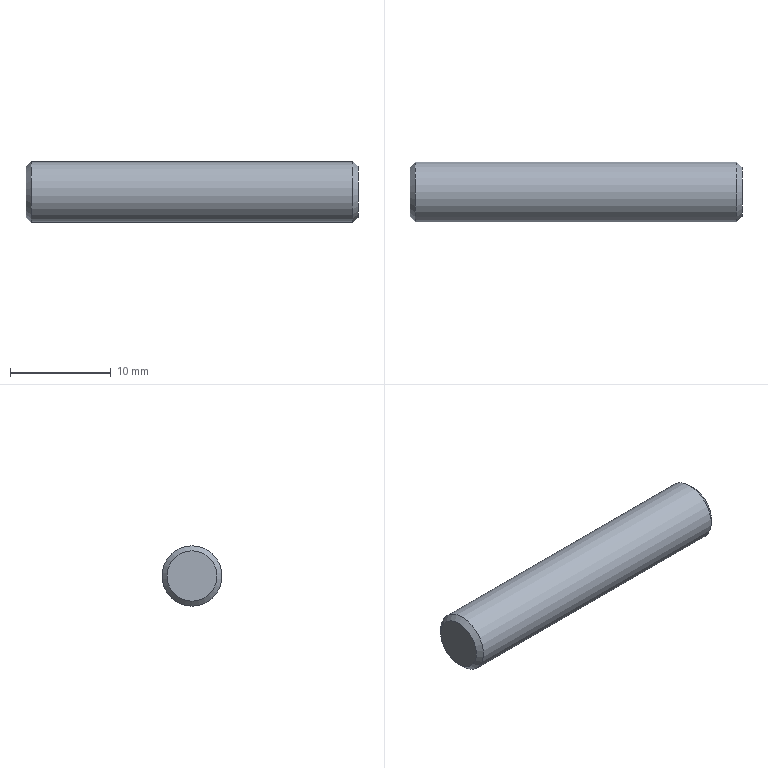Component | NX | STUD | 1 solid | 5 faces | box 33 x 6 x 6 mm | volume 929 mm3 | plane 2 | cone 2 | cylinder 1 | commonest cylinder face diameters 6 x1
STEP:
#1=CARTESIAN_POINT('',(0.,0.,0.));
#2=DIRECTION('',(0.,0.,1.));
#3=DIRECTION('',(1.,0.,0.));
#4=AXIS2_PLACEMENT_3D('',#1,#2,#3);
#5=CARTESIAN_POINT('',(-36.268,-25.,7.));
#6=VERTEX_POINT('',#5);
#7=CARTESIAN_POINT('',(-36.268,-25.,9.5));
#8=DIRECTION('',(1.,0.,0.));
#9=DIRECTION('',(0.,0.,-1.));
#10=AXIS2_PLACEMENT_3D('',#7,#8,#9);
#11=CIRCLE('',#10,2.5);
#12=CARTESIAN_POINT('',(-36.268,-25.,9.5));
#13=DIRECTION('',(1.,0.,0.));
#14=DIRECTION('',(0.,0.,-1.));
#15=AXIS2_PLACEMENT_3D('',#12,#13,#14);
#16=PLANE('',#15);
#17=CARTESIAN_POINT('',(0.,0.));
#18=DIRECTION('',(1.,0.));
#19=AXIS2_PLACEMENT_2D('',#17,#18);
#20=CIRCLE('',#19,2.5);
#21=(GEOMETRIC_REPRESENTATION_CONTEXT(2)PARAMETRIC_REPRESENTATION_CONTEXT()REPRESENTATION_CONTEXT('',''));
#22=DEFINITIONAL_REPRESENTATION('',(#20),#21);
#23=PCURVE('',#16,#22);
#24=CARTESIAN_POINT('',(-36.768,-25.,9.5));
#25=DIRECTION('',(-1.,0.,0.));
#26=DIRECTION('',(0.,0.,1.));
#27=AXIS2_PLACEMENT_3D('',#24,#25,#26);
#28=CONICAL_SURFACE('',#27,3.,0.7854);
#29=CARTESIAN_POINT('',(9.425,-0.5));
#30=DIRECTION('',(-1.,0.));
#31=VECTOR('',#30,1.);
#32=LINE('',#29,#31);
#33=(GEOMETRIC_REPRESENTATION_CONTEXT(2)PARAMETRIC_REPRESENTATION_CONTEXT()REPRESENTATION_CONTEXT('',''));
#34=DEFINITIONAL_REPRESENTATION('',(#32),#33);
#35=PCURVE('',#28,#34);
#36=SURFACE_CURVE('',#11,(#23,#35),.PCURVE_S1.);
#37=EDGE_CURVE('',#6,#6,#36,.T.);
#38=ORIENTED_EDGE('',*,*,#37,.T.);
#39=EDGE_LOOP('',(#38));
#40=FACE_BOUND('',#39,.T.);
#41=ADVANCED_FACE('',(#40),#16,.T.);
#42=CARTESIAN_POINT('',(-69.268,-25.,12.));
#43=VERTEX_POINT('',#42);
#44=CARTESIAN_POINT('',(-69.268,-25.,9.5));
#45=DIRECTION('',(-1.,0.,0.));
#46=DIRECTION('',(0.,0.,1.));
#47=AXIS2_PLACEMENT_3D('',#44,#45,#46);
#48=CIRCLE('',#47,2.5);
#49=CARTESIAN_POINT('',(-69.268,-25.,9.5));
#50=DIRECTION('',(-1.,0.,0.));
#51=DIRECTION('',(0.,0.,1.));
#52=AXIS2_PLACEMENT_3D('',#49,#50,#51);
#53=PLANE('',#52);
#54=CARTESIAN_POINT('',(0.,0.));
#55=DIRECTION('',(1.,0.));
#56=AXIS2_PLACEMENT_2D('',#54,#55);
#57=CIRCLE('',#56,2.5);
#58=(GEOMETRIC_REPRESENTATION_CONTEXT(2)PARAMETRIC_REPRESENTATION_CONTEXT()REPRESENTATION_CONTEXT('',''));
#59=DEFINITIONAL_REPRESENTATION('',(#57),#58);
#60=PCURVE('',#53,#59);
#61=CARTESIAN_POINT('',(-68.768,-25.,9.5));
#62=DIRECTION('',(1.,0.,0.));
#63=DIRECTION('',(0.,0.,-1.));
#64=AXIS2_PLACEMENT_3D('',#61,#62,#63);
#65=CONICAL_SURFACE('',#64,3.,0.7854);
#66=CARTESIAN_POINT('',(9.425,-0.5));
#67=DIRECTION('',(-1.,0.));
#68=VECTOR('',#67,1.);
#69=LINE('',#66,#68);
#70=(GEOMETRIC_REPRESENTATION_CONTEXT(2)PARAMETRIC_REPRESENTATION_CONTEXT()REPRESENTATION_CONTEXT('',''));
#71=DEFINITIONAL_REPRESENTATION('',(#69),#70);
#72=PCURVE('',#65,#71);
#73=SURFACE_CURVE('',#48,(#60,#72),.PCURVE_S1.);
#74=EDGE_CURVE('',#43,#43,#73,.T.);
#75=ORIENTED_EDGE('',*,*,#74,.T.);
#76=EDGE_LOOP('',(#75));
#77=FACE_BOUND('',#76,.T.);
#78=ADVANCED_FACE('',(#77),#53,.T.);
#79=CARTESIAN_POINT('',(-68.768,-25.,12.5));
#80=VERTEX_POINT('',#79);
#81=CARTESIAN_POINT('',(-68.768,-25.,6.5));
#82=VERTEX_POINT('',#81);
#83=CARTESIAN_POINT('',(-68.768,-25.,9.5));
#84=DIRECTION('',(1.,0.,0.));
#85=DIRECTION('',(0.,0.,1.));
#86=AXIS2_PLACEMENT_3D('',#83,#84,#85);
#87=CIRCLE('',#86,3.);
#88=CARTESIAN_POINT('',(-69.268,-25.,9.5));
#89=DIRECTION('',(1.,0.,0.));
#90=DIRECTION('',(0.,0.,-1.));
#91=AXIS2_PLACEMENT_3D('',#88,#89,#90);
#92=CYLINDRICAL_SURFACE('',#91,3.);
#93=CARTESIAN_POINT('',(3.142,0.5));
#94=DIRECTION('',(1.,0.));
#95=VECTOR('',#94,1.);
#96=LINE('',#93,#95);
#97=(GEOMETRIC_REPRESENTATION_CONTEXT(2)PARAMETRIC_REPRESENTATION_CONTEXT()REPRESENTATION_CONTEXT('',''));
#98=DEFINITIONAL_REPRESENTATION('',(#96),#97);
#99=PCURVE('',#92,#98);
#100=CARTESIAN_POINT('',(3.142,0.));
#101=DIRECTION('',(1.,0.));
#102=VECTOR('',#101,1.);
#103=LINE('',#100,#102);
#104=(GEOMETRIC_REPRESENTATION_CONTEXT(2)PARAMETRIC_REPRESENTATION_CONTEXT()REPRESENTATION_CONTEXT('',''));
#105=DEFINITIONAL_REPRESENTATION('',(#103),#104);
#106=PCURVE('',#65,#105);
#107=SURFACE_CURVE('',#87,(#99,#106),.PCURVE_S1.);
#108=EDGE_CURVE('',#80,#82,#107,.T.);
#109=ORIENTED_EDGE('',*,*,#108,.T.);
#110=CARTESIAN_POINT('',(-36.768,-25.,6.5));
#111=VERTEX_POINT('',#110);
#112=CARTESIAN_POINT('',(-68.768,-25.,6.5));
#113=CARTESIAN_POINT('',(-36.768,-25.,6.5));
#114=B_SPLINE_CURVE_WITH_KNOTS('',1,(#112,#113),.UNSPECIFIED.,.F.,.F.,(2,2),(0.5,32.5),.PIECEWISE_BEZIER_KNOTS.);
#115=CARTESIAN_POINT('',(6.283,0.));
#116=DIRECTION('',(0.,1.));
#117=VECTOR('',#116,1.);
#118=LINE('',#115,#117);
#119=(GEOMETRIC_REPRESENTATION_CONTEXT(2)PARAMETRIC_REPRESENTATION_CONTEXT()REPRESENTATION_CONTEXT('',''));
#120=DEFINITIONAL_REPRESENTATION('',(#118),#119);
#121=PCURVE('',#92,#120);
#122=CARTESIAN_POINT('',(0.,0.));
#123=DIRECTION('',(0.,1.));
#124=VECTOR('',#123,1.);
#125=LINE('',#122,#124);
#126=(GEOMETRIC_REPRESENTATION_CONTEXT(2)PARAMETRIC_REPRESENTATION_CONTEXT()REPRESENTATION_CONTEXT('',''));
#127=DEFINITIONAL_REPRESENTATION('',(#125),#126);
#128=PCURVE('',#92,#127);
#129=SEAM_CURVE('',#114,(#121,#128),.PCURVE_S1.);
#130=EDGE_CURVE('',#82,#111,#129,.T.);
#131=ORIENTED_EDGE('',*,*,#130,.T.);
#132=CARTESIAN_POINT('',(-36.768,-25.,9.5));
#133=DIRECTION('',(-1.,0.,0.));
#134=DIRECTION('',(0.,0.,-1.));
#135=AXIS2_PLACEMENT_3D('',#132,#133,#134);
#136=CIRCLE('',#135,3.);
#137=CARTESIAN_POINT('',(6.283,32.5));
#138=DIRECTION('',(-1.,0.));
#139=VECTOR('',#138,1.);
#140=LINE('',#137,#139);
#141=(GEOMETRIC_REPRESENTATION_CONTEXT(2)PARAMETRIC_REPRESENTATION_CONTEXT()REPRESENTATION_CONTEXT('',''));
#142=DEFINITIONAL_REPRESENTATION('',(#140),#141);
#143=PCURVE('',#92,#142);
#144=CARTESIAN_POINT('',(3.142,0.));
#145=DIRECTION('',(1.,0.));
#146=VECTOR('',#145,1.);
#147=LINE('',#144,#146);
#148=(GEOMETRIC_REPRESENTATION_CONTEXT(2)PARAMETRIC_REPRESENTATION_CONTEXT()REPRESENTATION_CONTEXT('',''));
#149=DEFINITIONAL_REPRESENTATION('',(#147),#148);
#150=PCURVE('',#28,#149);
#151=SURFACE_CURVE('',#136,(#143,#150),.PCURVE_S1.);
#152=EDGE_CURVE('',#111,#111,#151,.T.);
#153=ORIENTED_EDGE('',*,*,#152,.T.);
#154=ORIENTED_EDGE('',*,*,#130,.F.);
#155=CARTESIAN_POINT('',(-68.768,-25.,9.5));
#156=DIRECTION('',(1.,0.,0.));
#157=DIRECTION('',(0.,0.,1.));
#158=AXIS2_PLACEMENT_3D('',#155,#156,#157);
#159=CIRCLE('',#158,3.);
#160=CARTESIAN_POINT('',(-3.142,0.5));
#161=DIRECTION('',(1.,0.));
#162=VECTOR('',#161,1.);
#163=LINE('',#160,#162);
#164=(GEOMETRIC_REPRESENTATION_CONTEXT(2)PARAMETRIC_REPRESENTATION_CONTEXT()REPRESENTATION_CONTEXT('',''));
#165=DEFINITIONAL_REPRESENTATION('',(#163),#164);
#166=PCURVE('',#92,#165);
#167=CARTESIAN_POINT('',(3.142,0.));
#168=DIRECTION('',(1.,0.));
#169=VECTOR('',#168,1.);
#170=LINE('',#167,#169);
#171=(GEOMETRIC_REPRESENTATION_CONTEXT(2)PARAMETRIC_REPRESENTATION_CONTEXT()REPRESENTATION_CONTEXT('',''));
#172=DEFINITIONAL_REPRESENTATION('',(#170),#171);
#173=PCURVE('',#65,#172);
#174=SURFACE_CURVE('',#159,(#166,#173),.PCURVE_S1.);
#175=EDGE_CURVE('',#82,#80,#174,.T.);
#176=ORIENTED_EDGE('',*,*,#175,.T.);
#177=EDGE_LOOP('',(#109,#131,#153,#154,#176));
#178=FACE_BOUND('',#177,.T.);
#179=ADVANCED_FACE('',(#178),#92,.T.);
#180=ORIENTED_EDGE('',*,*,#74,.F.);
#181=CARTESIAN_POINT('',(-69.268,-25.,12.));
#182=CARTESIAN_POINT('',(-68.768,-25.,12.5));
#183=B_SPLINE_CURVE_WITH_KNOTS('',1,(#181,#182),.UNSPECIFIED.,.F.,.F.,(2,2),(-0.7071,0.),.PIECEWISE_BEZIER_KNOTS.);
#184=CARTESIAN_POINT('',(9.425,0.));
#185=DIRECTION('',(0.,1.));
#186=VECTOR('',#185,1.);
#187=LINE('',#184,#186);
#188=(GEOMETRIC_REPRESENTATION_CONTEXT(2)PARAMETRIC_REPRESENTATION_CONTEXT()REPRESENTATION_CONTEXT('',''));
#189=DEFINITIONAL_REPRESENTATION('',(#187),#188);
#190=PCURVE('',#65,#189);
#191=CARTESIAN_POINT('',(3.142,0.));
#192=DIRECTION('',(0.,1.));
#193=VECTOR('',#192,1.);
#194=LINE('',#191,#193);
#195=(GEOMETRIC_REPRESENTATION_CONTEXT(2)PARAMETRIC_REPRESENTATION_CONTEXT()REPRESENTATION_CONTEXT('',''));
#196=DEFINITIONAL_REPRESENTATION('',(#194),#195);
#197=PCURVE('',#65,#196);
#198=SEAM_CURVE('',#183,(#190,#197),.PCURVE_S1.);
#199=EDGE_CURVE('',#43,#80,#198,.T.);
#200=ORIENTED_EDGE('',*,*,#199,.T.);
#201=ORIENTED_EDGE('',*,*,#175,.F.);
#202=ORIENTED_EDGE('',*,*,#108,.F.);
#203=ORIENTED_EDGE('',*,*,#199,.F.);
#204=EDGE_LOOP('',(#180,#200,#201,#202,#203));
#205=FACE_BOUND('',#204,.T.);
#206=ADVANCED_FACE('',(#205),#65,.T.);
#207=ORIENTED_EDGE('',*,*,#37,.F.);
#208=CARTESIAN_POINT('',(-36.268,-25.,7.));
#209=CARTESIAN_POINT('',(-36.768,-25.,6.5));
#210=B_SPLINE_CURVE_WITH_KNOTS('',1,(#208,#209),.UNSPECIFIED.,.F.,.F.,(2,2),(-0.7071,0.),.PIECEWISE_BEZIER_KNOTS.);
#211=CARTESIAN_POINT('',(9.425,0.));
#212=DIRECTION('',(0.,1.));
#213=VECTOR('',#212,1.);
#214=LINE('',#211,#213);
#215=(GEOMETRIC_REPRESENTATION_CONTEXT(2)PARAMETRIC_REPRESENTATION_CONTEXT()REPRESENTATION_CONTEXT('',''));
#216=DEFINITIONAL_REPRESENTATION('',(#214),#215);
#217=PCURVE('',#28,#216);
#218=CARTESIAN_POINT('',(3.142,0.));
#219=DIRECTION('',(0.,1.));
#220=VECTOR('',#219,1.);
#221=LINE('',#218,#220);
#222=(GEOMETRIC_REPRESENTATION_CONTEXT(2)PARAMETRIC_REPRESENTATION_CONTEXT()REPRESENTATION_CONTEXT('',''));
#223=DEFINITIONAL_REPRESENTATION('',(#221),#222);
#224=PCURVE('',#28,#223);
#225=SEAM_CURVE('',#210,(#217,#224),.PCURVE_S1.);
#226=EDGE_CURVE('',#6,#111,#225,.T.);
#227=ORIENTED_EDGE('',*,*,#226,.T.);
#228=ORIENTED_EDGE('',*,*,#152,.F.);
#229=ORIENTED_EDGE('',*,*,#226,.F.);
#230=EDGE_LOOP('',(#207,#227,#228,#229));
#231=FACE_BOUND('',#230,.T.);
#232=ADVANCED_FACE('',(#231),#28,.T.);
#233=CLOSED_SHELL('',(#41,#78,#179,#206,#232));
#234=MANIFOLD_SOLID_BREP('',#233);
#235=(LENGTH_UNIT()NAMED_UNIT(*)SI_UNIT(.MILLI.,.METRE.));
#236=UNCERTAINTY_MEASURE_WITH_UNIT(LENGTH_MEASURE(0.00001),#235,'','');
#237=(NAMED_UNIT(*)PLANE_ANGLE_UNIT()SI_UNIT($,.RADIAN.));
#238=(NAMED_UNIT(*)SI_UNIT($,.STERADIAN.)SOLID_ANGLE_UNIT());
#239=(GEOMETRIC_REPRESENTATION_CONTEXT(3)GLOBAL_UNCERTAINTY_ASSIGNED_CONTEXT((#236))GLOBAL_UNIT_ASSIGNED_CONTEXT((#235,#237,#238))REPRESENTATION_CONTEXT('',''));
#240=ADVANCED_BREP_SHAPE_REPRESENTATION('',(#4,#234),#239);